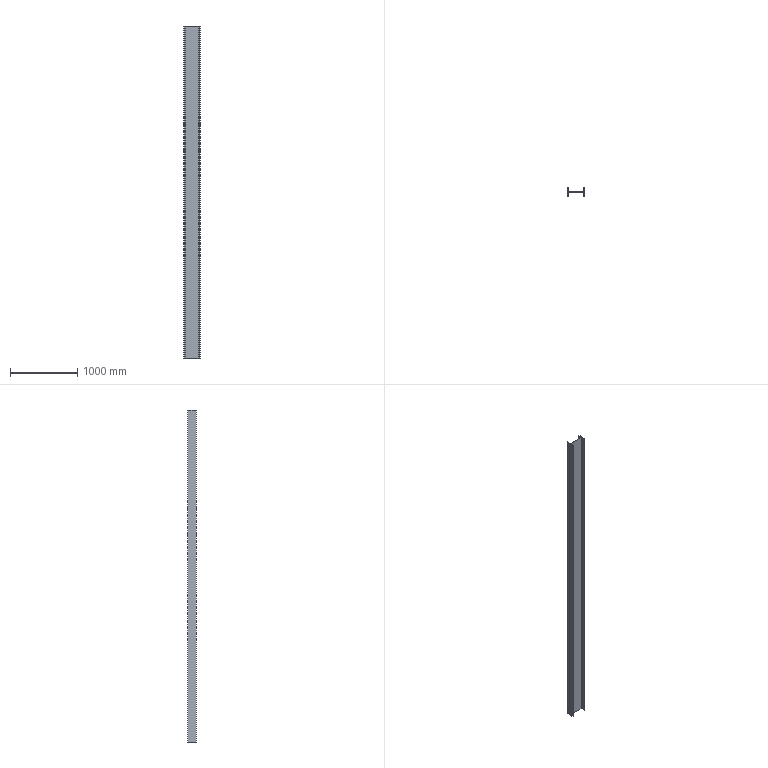Component | SolidWorks | H250X125-3800-4 | 1 solid | 18 faces | box 250 x 125 x 4930 mm | volume 18670259 mm3 | plane 14 | cylinder 4 | commonest cylinder face diameters 26 x4
STEP:
#1=COLOUR_RGB('',0.7922,0.8196,0.9333);
#2=FILL_AREA_STYLE_COLOUR('',#1);
#3=FILL_AREA_STYLE('',(#2));
#4=SURFACE_STYLE_FILL_AREA(#3);
#5=SURFACE_SIDE_STYLE('',(#4));
#6=SURFACE_STYLE_USAGE(.BOTH.,#5);
#7=PRESENTATION_STYLE_ASSIGNMENT((#6));
#8=CARTESIAN_POINT('',(71.651,-676.962,8.819));
#9=VERTEX_POINT('',#8);
#10=CARTESIAN_POINT('',(71.651,-676.962,202.913));
#11=VERTEX_POINT('',#10);
#12=CARTESIAN_POINT('',(71.651,-676.962,3.898));
#13=DIRECTION('',(0.,0.,1.));
#14=VECTOR('',#13,39.37);
#15=LINE('',#12,#14);
#16=EDGE_CURVE('',#9,#11,#15,.T.);
#17=ORIENTED_EDGE('',*,*,#16,.T.);
#18=CARTESIAN_POINT('',(71.651,-672.041,202.913));
#19=VERTEX_POINT('',#18);
#20=CARTESIAN_POINT('',(71.651,-672.041,202.913));
#21=DIRECTION('',(0.,1.,0.));
#22=VECTOR('',#21,39.37);
#23=LINE('',#20,#22);
#24=EDGE_CURVE('',#11,#19,#23,.T.);
#25=ORIENTED_EDGE('',*,*,#24,.T.);
#26=CARTESIAN_POINT('',(71.651,-672.041,8.819));
#27=VERTEX_POINT('',#26);
#28=CARTESIAN_POINT('',(71.651,-672.041,3.898));
#29=DIRECTION('',(0.,0.,1.));
#30=VECTOR('',#29,39.37);
#31=LINE('',#28,#30);
#32=EDGE_CURVE('',#27,#19,#31,.T.);
#33=ORIENTED_EDGE('',*,*,#32,.F.);
#34=CARTESIAN_POINT('',(71.651,-672.041,8.819));
#35=DIRECTION('',(0.,-1.,0.));
#36=VECTOR('',#35,39.37);
#37=LINE('',#34,#36);
#38=EDGE_CURVE('',#27,#9,#37,.T.);
#39=ORIENTED_EDGE('',*,*,#38,.T.);
#40=EDGE_LOOP('',(#17,#25,#33,#39));
#41=FACE_OUTER_BOUND('',#40,.T.);
#42=CARTESIAN_POINT('',(71.651,-672.041,3.898));
#43=DIRECTION('',(1.,0.,0.));
#44=DIRECTION('',(0.,0.,-1.));
#45=AXIS2_PLACEMENT_3D('',#42,#43,#44);
#46=PLANE('',#45);
#47=ADVANCED_FACE('',(#41),#46,.F.);
#48=ORIENTED_EDGE('',*,*,#32,.T.);
#49=CARTESIAN_POINT('',(72.005,-672.041,202.913));
#50=VERTEX_POINT('',#49);
#51=CARTESIAN_POINT('',(72.005,-672.041,202.913));
#52=DIRECTION('',(1.,0.,0.));
#53=VECTOR('',#52,39.37);
#54=LINE('',#51,#53);
#55=EDGE_CURVE('',#19,#50,#54,.T.);
#56=ORIENTED_EDGE('',*,*,#55,.T.);
#57=CARTESIAN_POINT('',(72.005,-672.041,8.819));
#58=VERTEX_POINT('',#57);
#59=CARTESIAN_POINT('',(72.005,-672.041,3.898));
#60=DIRECTION('',(0.,0.,1.));
#61=VECTOR('',#60,39.37);
#62=LINE('',#59,#61);
#63=EDGE_CURVE('',#58,#50,#62,.T.);
#64=ORIENTED_EDGE('',*,*,#63,.F.);
#65=CARTESIAN_POINT('',(72.005,-672.041,8.819));
#66=DIRECTION('',(-1.,0.,0.));
#67=VECTOR('',#66,39.37);
#68=LINE('',#65,#67);
#69=EDGE_CURVE('',#58,#27,#68,.T.);
#70=ORIENTED_EDGE('',*,*,#69,.T.);
#71=EDGE_LOOP('',(#48,#56,#64,#70));
#72=FACE_OUTER_BOUND('',#71,.T.);
#73=CARTESIAN_POINT('',(72.005,-672.041,3.898));
#74=DIRECTION('',(0.,-1.,0.));
#75=DIRECTION('',(-1.,0.,0.));
#76=AXIS2_PLACEMENT_3D('',#73,#74,#75);
#77=PLANE('',#76);
#78=ADVANCED_FACE('',(#72),#77,.F.);
#79=ORIENTED_EDGE('',*,*,#63,.T.);
#80=CARTESIAN_POINT('',(72.005,-673.872,202.913));
#81=VERTEX_POINT('',#80);
#82=CARTESIAN_POINT('',(72.005,-672.041,202.913));
#83=DIRECTION('',(0.,-1.,0.));
#84=VECTOR('',#83,39.37);
#85=LINE('',#82,#84);
#86=EDGE_CURVE('',#50,#81,#85,.T.);
#87=ORIENTED_EDGE('',*,*,#86,.T.);
#88=CARTESIAN_POINT('',(72.005,-673.872,8.819));
#89=VERTEX_POINT('',#88);
#90=CARTESIAN_POINT('',(72.005,-673.872,3.898));
#91=DIRECTION('',(0.,0.,1.));
#92=VECTOR('',#91,39.37);
#93=LINE('',#90,#92);
#94=EDGE_CURVE('',#89,#81,#93,.T.);
#95=ORIENTED_EDGE('',*,*,#94,.F.);
#96=CARTESIAN_POINT('',(72.005,-672.041,8.819));
#97=DIRECTION('',(-0.,1.,0.));
#98=VECTOR('',#97,39.37);
#99=LINE('',#96,#98);
#100=EDGE_CURVE('',#89,#58,#99,.T.);
#101=ORIENTED_EDGE('',*,*,#100,.T.);
#102=EDGE_LOOP('',(#79,#87,#95,#101));
#103=FACE_OUTER_BOUND('',#102,.T.);
#104=CARTESIAN_POINT('',(72.005,-672.041,3.898));
#105=DIRECTION('',(-1.,-0.,0.));
#106=DIRECTION('',(-0.,1.,0.));
#107=AXIS2_PLACEMENT_3D('',#104,#105,#106);
#108=PLANE('',#107);
#109=ADVANCED_FACE('',(#103),#108,.F.);
#110=ORIENTED_EDGE('',*,*,#94,.T.);
#111=CARTESIAN_POINT('',(72.517,-674.384,202.913));
#112=VERTEX_POINT('',#111);
#113=CARTESIAN_POINT('',(72.517,-673.872,202.913));
#114=DIRECTION('',(0.,0.,1.));
#115=DIRECTION('',(-1.,0.,0.));
#116=AXIS2_PLACEMENT_3D('',#113,#114,#115);
#117=CIRCLE('',#116,0.5118);
#118=EDGE_CURVE('',#81,#112,#117,.T.);
#119=ORIENTED_EDGE('',*,*,#118,.T.);
#120=CARTESIAN_POINT('',(72.517,-674.384,8.819));
#121=VERTEX_POINT('',#120);
#122=CARTESIAN_POINT('',(72.517,-674.384,3.898));
#123=DIRECTION('',(0.,0.,1.));
#124=VECTOR('',#123,39.37);
#125=LINE('',#122,#124);
#126=EDGE_CURVE('',#121,#112,#125,.T.);
#127=ORIENTED_EDGE('',*,*,#126,.F.);
#128=CARTESIAN_POINT('',(72.517,-673.872,8.819));
#129=DIRECTION('',(0.,0.,-1.));
#130=DIRECTION('',(1.,0.,0.));
#131=AXIS2_PLACEMENT_3D('',#128,#129,#130);
#132=CIRCLE('',#131,0.5118);
#133=EDGE_CURVE('',#121,#89,#132,.T.);
#134=ORIENTED_EDGE('',*,*,#133,.T.);
#135=EDGE_LOOP('',(#110,#119,#127,#134));
#136=FACE_OUTER_BOUND('',#135,.T.);
#137=CARTESIAN_POINT('',(72.517,-673.872,3.898));
#138=DIRECTION('',(0.,0.,1.));
#139=DIRECTION('',(1.,0.,0.));
#140=AXIS2_PLACEMENT_3D('',#137,#138,#139);
#141=CYLINDRICAL_SURFACE('',#140,0.5118);
#142=ADVANCED_FACE('',(#136),#141,.F.);
#143=ORIENTED_EDGE('',*,*,#126,.T.);
#144=CARTESIAN_POINT('',(80.627,-674.384,202.913));
#145=VERTEX_POINT('',#144);
#146=CARTESIAN_POINT('',(80.627,-674.384,202.913));
#147=DIRECTION('',(1.,-0.,0.));
#148=VECTOR('',#147,39.37);
#149=LINE('',#146,#148);
#150=EDGE_CURVE('',#112,#145,#149,.T.);
#151=ORIENTED_EDGE('',*,*,#150,.T.);
#152=CARTESIAN_POINT('',(80.627,-674.384,8.819));
#153=VERTEX_POINT('',#152);
#154=CARTESIAN_POINT('',(80.627,-674.384,3.898));
#155=DIRECTION('',(0.,0.,1.));
#156=VECTOR('',#155,39.37);
#157=LINE('',#154,#156);
#158=EDGE_CURVE('',#153,#145,#157,.T.);
#159=ORIENTED_EDGE('',*,*,#158,.F.);
#160=CARTESIAN_POINT('',(80.627,-674.384,8.819));
#161=DIRECTION('',(-1.,0.,0.));
#162=VECTOR('',#161,39.37);
#163=LINE('',#160,#162);
#164=EDGE_CURVE('',#153,#121,#163,.T.);
#165=ORIENTED_EDGE('',*,*,#164,.T.);
#166=EDGE_LOOP('',(#143,#151,#159,#165));
#167=FACE_OUTER_BOUND('',#166,.T.);
#168=CARTESIAN_POINT('',(80.627,-674.384,3.898));
#169=DIRECTION('',(-0.,-1.,0.));
#170=DIRECTION('',(-1.,0.,0.));
#171=AXIS2_PLACEMENT_3D('',#168,#169,#170);
#172=PLANE('',#171);
#173=ADVANCED_FACE('',(#167),#172,.F.);
#174=ORIENTED_EDGE('',*,*,#158,.T.);
#175=CARTESIAN_POINT('',(81.139,-673.872,202.913));
#176=VERTEX_POINT('',#175);
#177=CARTESIAN_POINT('',(80.627,-673.872,202.913));
#178=DIRECTION('',(0.,0.,1.));
#179=DIRECTION('',(-1.,0.,0.));
#180=AXIS2_PLACEMENT_3D('',#177,#178,#179);
#181=CIRCLE('',#180,0.5118);
#182=EDGE_CURVE('',#145,#176,#181,.T.);
#183=ORIENTED_EDGE('',*,*,#182,.T.);
#184=CARTESIAN_POINT('',(81.139,-673.872,8.819));
#185=VERTEX_POINT('',#184);
#186=CARTESIAN_POINT('',(81.139,-673.872,3.898));
#187=DIRECTION('',(0.,0.,1.));
#188=VECTOR('',#187,39.37);
#189=LINE('',#186,#188);
#190=EDGE_CURVE('',#185,#176,#189,.T.);
#191=ORIENTED_EDGE('',*,*,#190,.F.);
#192=CARTESIAN_POINT('',(80.627,-673.872,8.819));
#193=DIRECTION('',(0.,0.,-1.));
#194=DIRECTION('',(1.,0.,0.));
#195=AXIS2_PLACEMENT_3D('',#192,#193,#194);
#196=CIRCLE('',#195,0.5118);
#197=EDGE_CURVE('',#185,#153,#196,.T.);
#198=ORIENTED_EDGE('',*,*,#197,.T.);
#199=EDGE_LOOP('',(#174,#183,#191,#198));
#200=FACE_OUTER_BOUND('',#199,.T.);
#201=CARTESIAN_POINT('',(80.627,-673.872,3.898));
#202=DIRECTION('',(0.,0.,1.));
#203=DIRECTION('',(1.,0.,0.));
#204=AXIS2_PLACEMENT_3D('',#201,#202,#203);
#205=CYLINDRICAL_SURFACE('',#204,0.5118);
#206=ADVANCED_FACE('',(#200),#205,.F.);
#207=ORIENTED_EDGE('',*,*,#190,.T.);
#208=CARTESIAN_POINT('',(81.139,-672.041,202.913));
#209=VERTEX_POINT('',#208);
#210=CARTESIAN_POINT('',(81.139,-673.872,202.913));
#211=DIRECTION('',(0.,1.,0.));
#212=VECTOR('',#211,39.37);
#213=LINE('',#210,#212);
#214=EDGE_CURVE('',#176,#209,#213,.T.);
#215=ORIENTED_EDGE('',*,*,#214,.T.);
#216=CARTESIAN_POINT('',(81.139,-672.041,8.819));
#217=VERTEX_POINT('',#216);
#218=CARTESIAN_POINT('',(81.139,-672.041,3.898));
#219=DIRECTION('',(0.,0.,1.));
#220=VECTOR('',#219,39.37);
#221=LINE('',#218,#220);
#222=EDGE_CURVE('',#217,#209,#221,.T.);
#223=ORIENTED_EDGE('',*,*,#222,.F.);
#224=CARTESIAN_POINT('',(81.139,-673.872,8.819));
#225=DIRECTION('',(0.,-1.,0.));
#226=VECTOR('',#225,39.37);
#227=LINE('',#224,#226);
#228=EDGE_CURVE('',#217,#185,#227,.T.);
#229=ORIENTED_EDGE('',*,*,#228,.T.);
#230=EDGE_LOOP('',(#207,#215,#223,#229));
#231=FACE_OUTER_BOUND('',#230,.T.);
#232=CARTESIAN_POINT('',(81.139,-673.872,3.898));
#233=DIRECTION('',(1.,0.,0.));
#234=DIRECTION('',(0.,0.,-1.));
#235=AXIS2_PLACEMENT_3D('',#232,#233,#234);
#236=PLANE('',#235);
#237=ADVANCED_FACE('',(#231),#236,.F.);
#238=ORIENTED_EDGE('',*,*,#222,.T.);
#239=CARTESIAN_POINT('',(81.493,-672.041,202.913));
#240=VERTEX_POINT('',#239);
#241=CARTESIAN_POINT('',(81.493,-672.041,202.913));
#242=DIRECTION('',(1.,0.,0.));
#243=VECTOR('',#242,39.37);
#244=LINE('',#241,#243);
#245=EDGE_CURVE('',#209,#240,#244,.T.);
#246=ORIENTED_EDGE('',*,*,#245,.T.);
#247=CARTESIAN_POINT('',(81.493,-672.041,8.819));
#248=VERTEX_POINT('',#247);
#249=CARTESIAN_POINT('',(81.493,-672.041,3.898));
#250=DIRECTION('',(0.,0.,1.));
#251=VECTOR('',#250,39.37);
#252=LINE('',#249,#251);
#253=EDGE_CURVE('',#248,#240,#252,.T.);
#254=ORIENTED_EDGE('',*,*,#253,.F.);
#255=CARTESIAN_POINT('',(81.493,-672.041,8.819));
#256=DIRECTION('',(-1.,0.,0.));
#257=VECTOR('',#256,39.37);
#258=LINE('',#255,#257);
#259=EDGE_CURVE('',#248,#217,#258,.T.);
#260=ORIENTED_EDGE('',*,*,#259,.T.);
#261=EDGE_LOOP('',(#238,#246,#254,#260));
#262=FACE_OUTER_BOUND('',#261,.T.);
#263=CARTESIAN_POINT('',(81.493,-672.041,3.898));
#264=DIRECTION('',(0.,-1.,0.));
#265=DIRECTION('',(-1.,0.,0.));
#266=AXIS2_PLACEMENT_3D('',#263,#264,#265);
#267=PLANE('',#266);
#268=ADVANCED_FACE('',(#262),#267,.F.);
#269=ORIENTED_EDGE('',*,*,#253,.T.);
#270=CARTESIAN_POINT('',(81.493,-676.962,202.913));
#271=VERTEX_POINT('',#270);
#272=CARTESIAN_POINT('',(81.493,-676.962,202.913));
#273=DIRECTION('',(0.,-1.,0.));
#274=VECTOR('',#273,39.37);
#275=LINE('',#272,#274);
#276=EDGE_CURVE('',#240,#271,#275,.T.);
#277=ORIENTED_EDGE('',*,*,#276,.T.);
#278=CARTESIAN_POINT('',(81.493,-676.962,8.819));
#279=VERTEX_POINT('',#278);
#280=CARTESIAN_POINT('',(81.493,-676.962,3.898));
#281=DIRECTION('',(0.,0.,1.));
#282=VECTOR('',#281,39.37);
#283=LINE('',#280,#282);
#284=EDGE_CURVE('',#279,#271,#283,.T.);
#285=ORIENTED_EDGE('',*,*,#284,.F.);
#286=CARTESIAN_POINT('',(81.493,-676.962,8.819));
#287=DIRECTION('',(0.,1.,0.));
#288=VECTOR('',#287,39.37);
#289=LINE('',#286,#288);
#290=EDGE_CURVE('',#279,#248,#289,.T.);
#291=ORIENTED_EDGE('',*,*,#290,.T.);
#292=EDGE_LOOP('',(#269,#277,#285,#291));
#293=FACE_OUTER_BOUND('',#292,.T.);
#294=CARTESIAN_POINT('',(81.493,-676.962,3.898));
#295=DIRECTION('',(-1.,0.,0.));
#296=DIRECTION('',(0.,0.,1.));
#297=AXIS2_PLACEMENT_3D('',#294,#295,#296);
#298=PLANE('',#297);
#299=ADVANCED_FACE('',(#293),#298,.F.);
#300=ORIENTED_EDGE('',*,*,#284,.T.);
#301=CARTESIAN_POINT('',(81.139,-676.962,202.913));
#302=VERTEX_POINT('',#301);
#303=CARTESIAN_POINT('',(81.139,-676.962,202.913));
#304=DIRECTION('',(-1.,0.,0.));
#305=VECTOR('',#304,39.37);
#306=LINE('',#303,#305);
#307=EDGE_CURVE('',#271,#302,#306,.T.);
#308=ORIENTED_EDGE('',*,*,#307,.T.);
#309=CARTESIAN_POINT('',(81.139,-676.962,8.819));
#310=VERTEX_POINT('',#309);
#311=CARTESIAN_POINT('',(81.139,-676.962,3.898));
#312=DIRECTION('',(0.,0.,1.));
#313=VECTOR('',#312,39.37);
#314=LINE('',#311,#313);
#315=EDGE_CURVE('',#310,#302,#314,.T.);
#316=ORIENTED_EDGE('',*,*,#315,.F.);
#317=CARTESIAN_POINT('',(81.139,-676.962,8.819));
#318=DIRECTION('',(1.,0.,0.));
#319=VECTOR('',#318,39.37);
#320=LINE('',#317,#319);
#321=EDGE_CURVE('',#310,#279,#320,.T.);
#322=ORIENTED_EDGE('',*,*,#321,.T.);
#323=EDGE_LOOP('',(#300,#308,#316,#322));
#324=FACE_OUTER_BOUND('',#323,.T.);
#325=CARTESIAN_POINT('',(81.139,-676.962,3.898));
#326=DIRECTION('',(0.,1.,0.));
#327=DIRECTION('',(1.,0.,0.));
#328=AXIS2_PLACEMENT_3D('',#325,#326,#327);
#329=PLANE('',#328);
#330=ADVANCED_FACE('',(#324),#329,.F.);
#331=ORIENTED_EDGE('',*,*,#315,.T.);
#332=CARTESIAN_POINT('',(81.139,-675.132,202.913));
#333=VERTEX_POINT('',#332);
#334=CARTESIAN_POINT('',(81.139,-676.962,202.913));
#335=DIRECTION('',(0.,1.,0.));
#336=VECTOR('',#335,39.37);
#337=LINE('',#334,#336);
#338=EDGE_CURVE('',#302,#333,#337,.T.);
#339=ORIENTED_EDGE('',*,*,#338,.T.);
#340=CARTESIAN_POINT('',(81.139,-675.132,8.819));
#341=VERTEX_POINT('',#340);
#342=CARTESIAN_POINT('',(81.139,-675.132,3.898));
#343=DIRECTION('',(0.,0.,1.));
#344=VECTOR('',#343,39.37);
#345=LINE('',#342,#344);
#346=EDGE_CURVE('',#341,#333,#345,.T.);
#347=ORIENTED_EDGE('',*,*,#346,.F.);
#348=CARTESIAN_POINT('',(81.139,-676.962,8.819));
#349=DIRECTION('',(0.,-1.,0.));
#350=VECTOR('',#349,39.37);
#351=LINE('',#348,#350);
#352=EDGE_CURVE('',#341,#310,#351,.T.);
#353=ORIENTED_EDGE('',*,*,#352,.T.);
#354=EDGE_LOOP('',(#331,#339,#347,#353));
#355=FACE_OUTER_BOUND('',#354,.T.);
#356=CARTESIAN_POINT('',(81.139,-676.962,3.898));
#357=DIRECTION('',(1.,0.,0.));
#358=DIRECTION('',(0.,0.,-1.));
#359=AXIS2_PLACEMENT_3D('',#356,#357,#358);
#360=PLANE('',#359);
#361=ADVANCED_FACE('',(#355),#360,.F.);
#362=ORIENTED_EDGE('',*,*,#346,.T.);
#363=CARTESIAN_POINT('',(80.627,-674.62,202.913));
#364=VERTEX_POINT('',#363);
#365=CARTESIAN_POINT('',(80.627,-675.132,202.913));
#366=DIRECTION('',(0.,0.,1.));
#367=DIRECTION('',(-1.,0.,0.));
#368=AXIS2_PLACEMENT_3D('',#365,#366,#367);
#369=CIRCLE('',#368,0.5118);
#370=EDGE_CURVE('',#333,#364,#369,.T.);
#371=ORIENTED_EDGE('',*,*,#370,.T.);
#372=CARTESIAN_POINT('',(80.627,-674.62,8.819));
#373=VERTEX_POINT('',#372);
#374=CARTESIAN_POINT('',(80.627,-674.62,3.898));
#375=DIRECTION('',(0.,0.,1.));
#376=VECTOR('',#375,39.37);
#377=LINE('',#374,#376);
#378=EDGE_CURVE('',#373,#364,#377,.T.);
#379=ORIENTED_EDGE('',*,*,#378,.F.);
#380=CARTESIAN_POINT('',(80.627,-675.132,8.819));
#381=DIRECTION('',(0.,0.,-1.));
#382=DIRECTION('',(1.,0.,0.));
#383=AXIS2_PLACEMENT_3D('',#380,#381,#382);
#384=CIRCLE('',#383,0.5118);
#385=EDGE_CURVE('',#373,#341,#384,.T.);
#386=ORIENTED_EDGE('',*,*,#385,.T.);
#387=EDGE_LOOP('',(#362,#371,#379,#386));
#388=FACE_OUTER_BOUND('',#387,.T.);
#389=CARTESIAN_POINT('',(80.627,-675.132,3.898));
#390=DIRECTION('',(0.,0.,1.));
#391=DIRECTION('',(1.,0.,0.));
#392=AXIS2_PLACEMENT_3D('',#389,#390,#391);
#393=CYLINDRICAL_SURFACE('',#392,0.5118);
#394=ADVANCED_FACE('',(#388),#393,.F.);
#395=ORIENTED_EDGE('',*,*,#378,.T.);
#396=CARTESIAN_POINT('',(72.517,-674.62,202.913));
#397=VERTEX_POINT('',#396);
#398=CARTESIAN_POINT('',(72.517,-674.62,202.913));
#399=DIRECTION('',(-1.,0.,0.));
#400=VECTOR('',#399,39.37);
#401=LINE('',#398,#400);
#402=EDGE_CURVE('',#364,#397,#401,.T.);
#403=ORIENTED_EDGE('',*,*,#402,.T.);
#404=CARTESIAN_POINT('',(72.517,-674.62,8.819));
#405=VERTEX_POINT('',#404);
#406=CARTESIAN_POINT('',(72.517,-674.62,3.898));
#407=DIRECTION('',(0.,0.,1.));
#408=VECTOR('',#407,39.37);
#409=LINE('',#406,#408);
#410=EDGE_CURVE('',#405,#397,#409,.T.);
#411=ORIENTED_EDGE('',*,*,#410,.F.);
#412=CARTESIAN_POINT('',(72.517,-674.62,8.819));
#413=DIRECTION('',(1.,-0.,0.));
#414=VECTOR('',#413,39.37);
#415=LINE('',#412,#414);
#416=EDGE_CURVE('',#405,#373,#415,.T.);
#417=ORIENTED_EDGE('',*,*,#416,.T.);
#418=EDGE_LOOP('',(#395,#403,#411,#417));
#419=FACE_OUTER_BOUND('',#418,.T.);
#420=CARTESIAN_POINT('',(72.517,-674.62,3.898));
#421=DIRECTION('',(0.,1.,0.));
#422=DIRECTION('',(1.,-0.,0.));
#423=AXIS2_PLACEMENT_3D('',#420,#421,#422);
#424=PLANE('',#423);
#425=ADVANCED_FACE('',(#419),#424,.F.);
#426=ORIENTED_EDGE('',*,*,#410,.T.);
#427=CARTESIAN_POINT('',(72.005,-675.132,202.913));
#428=VERTEX_POINT('',#427);
#429=CARTESIAN_POINT('',(72.517,-675.132,202.913));
#430=DIRECTION('',(0.,0.,1.));
#431=DIRECTION('',(-1.,0.,0.));
#432=AXIS2_PLACEMENT_3D('',#429,#430,#431);
#433=CIRCLE('',#432,0.5118);
#434=EDGE_CURVE('',#397,#428,#433,.T.);
#435=ORIENTED_EDGE('',*,*,#434,.T.);
#436=CARTESIAN_POINT('',(72.005,-675.132,8.819));
#437=VERTEX_POINT('',#436);
#438=CARTESIAN_POINT('',(72.005,-675.132,3.898));
#439=DIRECTION('',(0.,0.,1.));
#440=VECTOR('',#439,39.37);
#441=LINE('',#438,#440);
#442=EDGE_CURVE('',#437,#428,#441,.T.);
#443=ORIENTED_EDGE('',*,*,#442,.F.);
#444=CARTESIAN_POINT('',(72.517,-675.132,8.819));
#445=DIRECTION('',(0.,0.,-1.));
#446=DIRECTION('',(1.,0.,0.));
#447=AXIS2_PLACEMENT_3D('',#444,#445,#446);
#448=CIRCLE('',#447,0.5118);
#449=EDGE_CURVE('',#437,#405,#448,.T.);
#450=ORIENTED_EDGE('',*,*,#449,.T.);
#451=EDGE_LOOP('',(#426,#435,#443,#450));
#452=FACE_OUTER_BOUND('',#451,.T.);
#453=CARTESIAN_POINT('',(72.517,-675.132,3.898));
#454=DIRECTION('',(0.,0.,1.));
#455=DIRECTION('',(1.,0.,0.));
#456=AXIS2_PLACEMENT_3D('',#453,#454,#455);
#457=CYLINDRICAL_SURFACE('',#456,0.5118);
#458=ADVANCED_FACE('',(#452),#457,.F.);
#459=ORIENTED_EDGE('',*,*,#442,.T.);
#460=CARTESIAN_POINT('',(72.005,-676.962,202.913));
#461=VERTEX_POINT('',#460);
#462=CARTESIAN_POINT('',(72.005,-675.132,202.913));
#463=DIRECTION('',(-0.,-1.,0.));
#464=VECTOR('',#463,39.37);
#465=LINE('',#462,#464);
#466=EDGE_CURVE('',#428,#461,#465,.T.);
#467=ORIENTED_EDGE('',*,*,#466,.T.);
#468=CARTESIAN_POINT('',(72.005,-676.962,8.819));
#469=VERTEX_POINT('',#468);
#470=CARTESIAN_POINT('',(72.005,-676.962,3.898));
#471=DIRECTION('',(0.,0.,1.));
#472=VECTOR('',#471,39.37);
#473=LINE('',#470,#472);
#474=EDGE_CURVE('',#469,#461,#473,.T.);
#475=ORIENTED_EDGE('',*,*,#474,.F.);
#476=CARTESIAN_POINT('',(72.005,-675.132,8.819));
#477=DIRECTION('',(0.,1.,0.));
#478=VECTOR('',#477,39.37);
#479=LINE('',#476,#478);
#480=EDGE_CURVE('',#469,#437,#479,.T.);
#481=ORIENTED_EDGE('',*,*,#480,.T.);
#482=EDGE_LOOP('',(#459,#467,#475,#481));
#483=FACE_OUTER_BOUND('',#482,.T.);
#484=CARTESIAN_POINT('',(72.005,-675.132,3.898));
#485=DIRECTION('',(-1.,0.,0.));
#486=DIRECTION('',(0.,1.,0.));
#487=AXIS2_PLACEMENT_3D('',#484,#485,#486);
#488=PLANE('',#487);
#489=ADVANCED_FACE('',(#483),#488,.F.);
#490=ORIENTED_EDGE('',*,*,#474,.T.);
#491=CARTESIAN_POINT('',(71.651,-676.962,202.913));
#492=DIRECTION('',(-1.,0.,0.));
#493=VECTOR('',#492,39.37);
#494=LINE('',#491,#493);
#495=EDGE_CURVE('',#461,#11,#494,.T.);
#496=ORIENTED_EDGE('',*,*,#495,.T.);
#497=ORIENTED_EDGE('',*,*,#16,.F.);
#498=CARTESIAN_POINT('',(71.651,-676.962,8.819));
#499=DIRECTION('',(1.,0.,0.));
#500=VECTOR('',#499,39.37);
#501=LINE('',#498,#500);
#502=EDGE_CURVE('',#9,#469,#501,.T.);
#503=ORIENTED_EDGE('',*,*,#502,.T.);
#504=EDGE_LOOP('',(#490,#496,#497,#503));
#505=FACE_OUTER_BOUND('',#504,.T.);
#506=CARTESIAN_POINT('',(71.651,-676.962,3.898));
#507=DIRECTION('',(0.,1.,0.));
#508=DIRECTION('',(1.,0.,0.));
#509=AXIS2_PLACEMENT_3D('',#506,#507,#508);
#510=PLANE('',#509);
#511=ADVANCED_FACE('',(#505),#510,.F.);
#512=ORIENTED_EDGE('',*,*,#69,.F.);
#513=ORIENTED_EDGE('',*,*,#100,.F.);
#514=ORIENTED_EDGE('',*,*,#133,.F.);
#515=ORIENTED_EDGE('',*,*,#164,.F.);
#516=ORIENTED_EDGE('',*,*,#197,.F.);
#517=ORIENTED_EDGE('',*,*,#228,.F.);
#518=ORIENTED_EDGE('',*,*,#259,.F.);
#519=ORIENTED_EDGE('',*,*,#290,.F.);
#520=ORIENTED_EDGE('',*,*,#321,.F.);
#521=ORIENTED_EDGE('',*,*,#352,.F.);
#522=ORIENTED_EDGE('',*,*,#385,.F.);
#523=ORIENTED_EDGE('',*,*,#416,.F.);
#524=ORIENTED_EDGE('',*,*,#449,.F.);
#525=ORIENTED_EDGE('',*,*,#480,.F.);
#526=ORIENTED_EDGE('',*,*,#502,.F.);
#527=ORIENTED_EDGE('',*,*,#38,.F.);
#528=EDGE_LOOP('',(#512,#513,#514,#515,#516,#517,#518,#519,#520,#521,#522,#523,#524,#525,#526,#527));
#529=FACE_OUTER_BOUND('',#528,.T.);
#530=CARTESIAN_POINT('',(-68.113,-917.323,8.819));
#531=DIRECTION('',(0.,0.,1.));
#532=DIRECTION('',(1.,0.,0.));
#533=AXIS2_PLACEMENT_3D('',#530,#531,#532);
#534=PLANE('',#533);
#535=ADVANCED_FACE('',(#529),#534,.F.);
#536=ORIENTED_EDGE('',*,*,#495,.F.);
#537=ORIENTED_EDGE('',*,*,#466,.F.);
#538=ORIENTED_EDGE('',*,*,#434,.F.);
#539=ORIENTED_EDGE('',*,*,#402,.F.);
#540=ORIENTED_EDGE('',*,*,#370,.F.);
#541=ORIENTED_EDGE('',*,*,#338,.F.);
#542=ORIENTED_EDGE('',*,*,#307,.F.);
#543=ORIENTED_EDGE('',*,*,#276,.F.);
#544=ORIENTED_EDGE('',*,*,#245,.F.);
#545=ORIENTED_EDGE('',*,*,#214,.F.);
#546=ORIENTED_EDGE('',*,*,#182,.F.);
#547=ORIENTED_EDGE('',*,*,#150,.F.);
#548=ORIENTED_EDGE('',*,*,#118,.F.);
#549=ORIENTED_EDGE('',*,*,#86,.F.);
#550=ORIENTED_EDGE('',*,*,#55,.F.);
#551=ORIENTED_EDGE('',*,*,#24,.F.);
#552=EDGE_LOOP('',(#536,#537,#538,#539,#540,#541,#542,#543,#544,#545,#546,#547,#548,#549,#550,#551));
#553=FACE_OUTER_BOUND('',#552,.T.);
#554=CARTESIAN_POINT('',(-68.113,-917.323,202.913));
#555=DIRECTION('',(0.,0.,-1.));
#556=DIRECTION('',(-1.,0.,0.));
#557=AXIS2_PLACEMENT_3D('',#554,#555,#556);
#558=PLANE('',#557);
#559=ADVANCED_FACE('',(#553),#558,.F.);
#560=CLOSED_SHELL('',(#47,#78,#109,#142,#173,#206,#237,#268,#299,#330,#361,#394,#425,#458,#489,#511,#535,#559));
#561=MANIFOLD_SOLID_BREP('',#560);
#562=STYLED_ITEM('',(#7),#561);
#563=(LENGTH_UNIT()NAMED_UNIT(*)SI_UNIT($,.METRE.));
#564=LENGTH_MEASURE_WITH_UNIT(LENGTH_MEASURE(0.0254),#563);
#565=DIMENSIONAL_EXPONENTS(1.,0.,0.,0.,0.,0.,0.);
#566=(CONVERSION_BASED_UNIT('',#564)LENGTH_UNIT()NAMED_UNIT(#565));
#567=UNCERTAINTY_MEASURE_WITH_UNIT(LENGTH_MEASURE(0.00001),#566,'','');
#568=(NAMED_UNIT(*)PLANE_ANGLE_UNIT()SI_UNIT($,.RADIAN.));
#569=(NAMED_UNIT(*)SI_UNIT($,.STERADIAN.)SOLID_ANGLE_UNIT());
#570=(GEOMETRIC_REPRESENTATION_CONTEXT(3)GLOBAL_UNCERTAINTY_ASSIGNED_CONTEXT((#567))GLOBAL_UNIT_ASSIGNED_CONTEXT((#566,#568,#569))REPRESENTATION_CONTEXT('',''));
#571=MECHANICAL_DESIGN_GEOMETRIC_PRESENTATION_REPRESENTATION('',(#562),#570);
#572=CARTESIAN_POINT('',(0.,0.,0.));
#573=DIRECTION('',(0.,0.,1.));
#574=DIRECTION('',(1.,0.,0.));
#575=AXIS2_PLACEMENT_3D('',#572,#573,#574);
#576=(LENGTH_UNIT()NAMED_UNIT(*)SI_UNIT($,.METRE.));
#577=LENGTH_MEASURE_WITH_UNIT(LENGTH_MEASURE(0.0254),#576);
#578=DIMENSIONAL_EXPONENTS(1.,0.,0.,0.,0.,0.,0.);
#579=(CONVERSION_BASED_UNIT('',#577)LENGTH_UNIT()NAMED_UNIT(#578));
#580=UNCERTAINTY_MEASURE_WITH_UNIT(LENGTH_MEASURE(0.00001),#579,'','');
#581=(NAMED_UNIT(*)PLANE_ANGLE_UNIT()SI_UNIT($,.RADIAN.));
#582=(NAMED_UNIT(*)SI_UNIT($,.STERADIAN.)SOLID_ANGLE_UNIT());
#583=(GEOMETRIC_REPRESENTATION_CONTEXT(3)GLOBAL_UNCERTAINTY_ASSIGNED_CONTEXT((#580))GLOBAL_UNIT_ASSIGNED_CONTEXT((#579,#581,#582))REPRESENTATION_CONTEXT('',''));
#584=ADVANCED_BREP_SHAPE_REPRESENTATION('',(#561,#575),#583);
#585=PRESENTATION_LAYER_ASSIGNMENT('','',(#562));